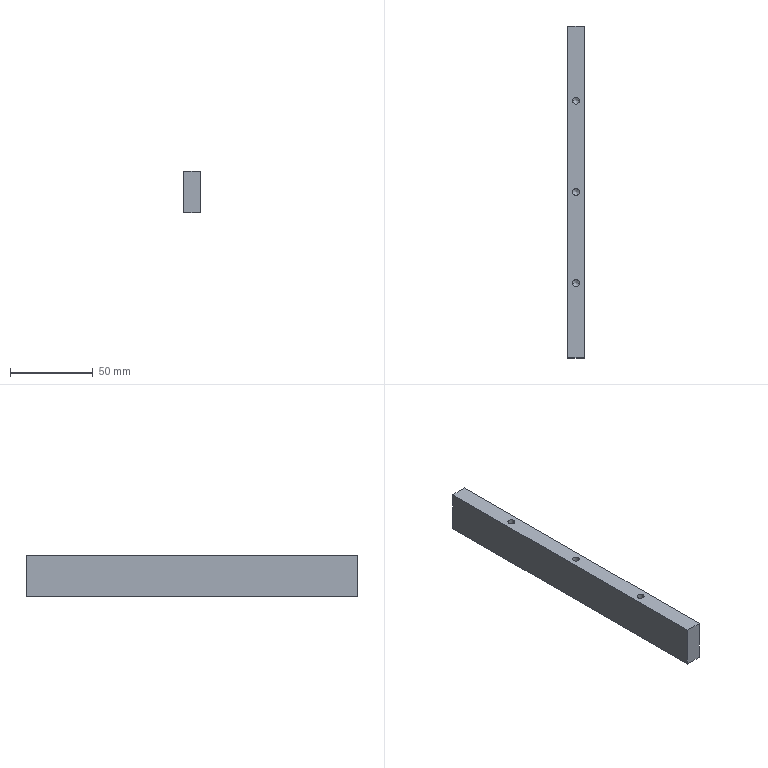Component | SolidWorks | P-SLJ-001-001-1 | 1 solid | 18 faces | box 10 x 200 x 25 mm | volume 49401 mm3 | cylinder 6 | cone 6 | plane 6 | commonest cylinder face diameters 4.2 x6 | material 45#
build123d program:
from build123d import *

# Parameters (mm, degrees)
SKETCH1_W             = 10
SKETCH1_H             = 200
EXTRUDE1_DEPTH        = 12.5
M5_TAPPED_HOLE1_D     = 4.2
M5_TAPPED_HOLE1_DEPTH = 14
M5_TAPPED_HOLE1_TIP   = 1.262


with BuildPart() as part:
    # Sketch1 → Extrude1 (new, symmetric)
    with BuildSketch(Plane(origin=(0, 0, 0), x_dir=(0, 0, -1), z_dir=(1, 0, 0))):
        Rectangle(SKETCH1_W, SKETCH1_H)
    extrude(amount=EXTRUDE1_DEPTH, both=True)

    # M5 Tapped Hole1
    with Locations(Plane.ZY.offset(12.5)):
        with Locations((0, 55), (0, 0), (0, -55)):
            Hole(M5_TAPPED_HOLE1_D / 2, depth=M5_TAPPED_HOLE1_DEPTH)
            with Locations((0, 0, -(M5_TAPPED_HOLE1_DEPTH + M5_TAPPED_HOLE1_TIP / 2))):  # 118° drill point
                Cone(0, M5_TAPPED_HOLE1_D / 2, M5_TAPPED_HOLE1_TIP, mode=Mode.SUBTRACT)


solid = part.part

# Placed as in the assembly
solid = solid.moved(Location((221.5, 0, 1213.134), (0, 90, 0)))
STEP:
#1=COLOUR_RGB('',0.7922,0.8196,0.9333);
#2=FILL_AREA_STYLE_COLOUR('',#1);
#3=FILL_AREA_STYLE('',(#2));
#4=SURFACE_STYLE_FILL_AREA(#3);
#5=SURFACE_SIDE_STYLE('',(#4));
#6=SURFACE_STYLE_USAGE(.BOTH.,#5);
#7=PRESENTATION_STYLE_ASSIGNMENT((#6));
#8=CARTESIAN_POINT('',(8.638,2.165,47.702));
#9=VERTEX_POINT('',#8);
#10=CARTESIAN_POINT('',(8.803,2.165,47.702));
#11=VERTEX_POINT('',#10);
#12=CARTESIAN_POINT('',(8.72,2.165,47.702));
#13=DIRECTION('',(0.,0.,1.));
#14=DIRECTION('',(1.,0.,0.));
#15=AXIS2_PLACEMENT_3D('',#12,#13,#14);
#16=CIRCLE('',#15,0.08268);
#17=EDGE_CURVE('',#9,#11,#16,.T.);
#18=ORIENTED_EDGE('',*,*,#17,.F.);
#19=CARTESIAN_POINT('',(8.638,2.165,48.253));
#20=VERTEX_POINT('',#19);
#21=CARTESIAN_POINT('',(8.638,2.165,48.253));
#22=DIRECTION('',(0.,0.,1.));
#23=VECTOR('',#22,39.37);
#24=LINE('',#21,#23);
#25=EDGE_CURVE('',#9,#20,#24,.T.);
#26=ORIENTED_EDGE('',*,*,#25,.T.);
#27=CARTESIAN_POINT('',(8.803,2.165,48.253));
#28=VERTEX_POINT('',#27);
#29=CARTESIAN_POINT('',(8.72,2.165,48.253));
#30=DIRECTION('',(0.,0.,1.));
#31=DIRECTION('',(1.,0.,0.));
#32=AXIS2_PLACEMENT_3D('',#29,#30,#31);
#33=CIRCLE('',#32,0.08268);
#34=EDGE_CURVE('',#20,#28,#33,.T.);
#35=ORIENTED_EDGE('',*,*,#34,.T.);
#36=CARTESIAN_POINT('',(8.803,2.165,48.253));
#37=DIRECTION('',(0.,0.,1.));
#38=VECTOR('',#37,39.37);
#39=LINE('',#36,#38);
#40=EDGE_CURVE('',#11,#28,#39,.T.);
#41=ORIENTED_EDGE('',*,*,#40,.F.);
#42=EDGE_LOOP('',(#18,#26,#35,#41));
#43=FACE_OUTER_BOUND('',#42,.T.);
#44=CARTESIAN_POINT('',(8.72,2.165,48.253));
#45=DIRECTION('',(0.,0.,1.));
#46=DIRECTION('',(1.,0.,0.));
#47=AXIS2_PLACEMENT_3D('',#44,#45,#46);
#48=CYLINDRICAL_SURFACE('',#47,0.08268);
#49=ADVANCED_FACE('',(#43),#48,.F.);
#50=CARTESIAN_POINT('',(8.72,2.165,47.652));
#51=VERTEX_POINT('',#50);
#52=CARTESIAN_POINT('',(8.803,2.165,47.702));
#53=DIRECTION('',(0.8572,-0.,0.515));
#54=VECTOR('',#53,39.37);
#55=LINE('',#52,#54);
#56=EDGE_CURVE('',#51,#11,#55,.T.);
#57=ORIENTED_EDGE('',*,*,#56,.F.);
#58=CARTESIAN_POINT('',(8.638,2.165,47.702));
#59=DIRECTION('',(-0.8572,0.,0.515));
#60=VECTOR('',#59,39.37);
#61=LINE('',#58,#60);
#62=EDGE_CURVE('',#51,#9,#61,.T.);
#63=ORIENTED_EDGE('',*,*,#62,.T.);
#64=ORIENTED_EDGE('',*,*,#17,.T.);
#65=EDGE_LOOP('',(#57,#63,#64));
#66=FACE_OUTER_BOUND('',#65,.T.);
#67=CARTESIAN_POINT('',(8.72,2.165,47.702));
#68=DIRECTION('',(0.,0.,1.));
#69=DIRECTION('',(1.,0.,0.));
#70=AXIS2_PLACEMENT_3D('',#67,#68,#69);
#71=CONICAL_SURFACE('',#70,0.08268,1.03);
#72=ADVANCED_FACE('',(#66),#71,.F.);
#73=CARTESIAN_POINT('',(8.638,-0.,47.702));
#74=VERTEX_POINT('',#73);
#75=CARTESIAN_POINT('',(8.803,-0.,47.702));
#76=VERTEX_POINT('',#75);
#77=CARTESIAN_POINT('',(8.72,-0.,47.702));
#78=DIRECTION('',(0.,0.,1.));
#79=DIRECTION('',(1.,-0.,0.));
#80=AXIS2_PLACEMENT_3D('',#77,#78,#79);
#81=CIRCLE('',#80,0.08268);
#82=EDGE_CURVE('',#74,#76,#81,.T.);
#83=ORIENTED_EDGE('',*,*,#82,.F.);
#84=CARTESIAN_POINT('',(8.638,-0.,48.253));
#85=VERTEX_POINT('',#84);
#86=CARTESIAN_POINT('',(8.638,-0.,48.253));
#87=DIRECTION('',(0.,0.,1.));
#88=VECTOR('',#87,39.37);
#89=LINE('',#86,#88);
#90=EDGE_CURVE('',#74,#85,#89,.T.);
#91=ORIENTED_EDGE('',*,*,#90,.T.);
#92=CARTESIAN_POINT('',(8.803,-0.,48.253));
#93=VERTEX_POINT('',#92);
#94=CARTESIAN_POINT('',(8.72,-0.,48.253));
#95=DIRECTION('',(0.,0.,1.));
#96=DIRECTION('',(1.,-0.,0.));
#97=AXIS2_PLACEMENT_3D('',#94,#95,#96);
#98=CIRCLE('',#97,0.08268);
#99=EDGE_CURVE('',#85,#93,#98,.T.);
#100=ORIENTED_EDGE('',*,*,#99,.T.);
#101=CARTESIAN_POINT('',(8.803,-0.,48.253));
#102=DIRECTION('',(0.,0.,1.));
#103=VECTOR('',#102,39.37);
#104=LINE('',#101,#103);
#105=EDGE_CURVE('',#76,#93,#104,.T.);
#106=ORIENTED_EDGE('',*,*,#105,.F.);
#107=EDGE_LOOP('',(#83,#91,#100,#106));
#108=FACE_OUTER_BOUND('',#107,.T.);
#109=CARTESIAN_POINT('',(8.72,-0.,48.253));
#110=DIRECTION('',(0.,0.,1.));
#111=DIRECTION('',(1.,-0.,0.));
#112=AXIS2_PLACEMENT_3D('',#109,#110,#111);
#113=CYLINDRICAL_SURFACE('',#112,0.08268);
#114=ADVANCED_FACE('',(#108),#113,.F.);
#115=CARTESIAN_POINT('',(8.72,-0.,47.652));
#116=VERTEX_POINT('',#115);
#117=CARTESIAN_POINT('',(8.803,-0.,47.702));
#118=DIRECTION('',(0.8572,-0.,0.515));
#119=VECTOR('',#118,39.37);
#120=LINE('',#117,#119);
#121=EDGE_CURVE('',#116,#76,#120,.T.);
#122=ORIENTED_EDGE('',*,*,#121,.F.);
#123=CARTESIAN_POINT('',(8.638,-0.,47.702));
#124=DIRECTION('',(-0.8572,0.,0.515));
#125=VECTOR('',#124,39.37);
#126=LINE('',#123,#125);
#127=EDGE_CURVE('',#116,#74,#126,.T.);
#128=ORIENTED_EDGE('',*,*,#127,.T.);
#129=ORIENTED_EDGE('',*,*,#82,.T.);
#130=EDGE_LOOP('',(#122,#128,#129));
#131=FACE_OUTER_BOUND('',#130,.T.);
#132=CARTESIAN_POINT('',(8.72,-0.,47.702));
#133=DIRECTION('',(0.,0.,1.));
#134=DIRECTION('',(1.,-0.,0.));
#135=AXIS2_PLACEMENT_3D('',#132,#133,#134);
#136=CONICAL_SURFACE('',#135,0.08268,1.03);
#137=ADVANCED_FACE('',(#131),#136,.F.);
#138=CARTESIAN_POINT('',(8.638,-2.165,47.702));
#139=VERTEX_POINT('',#138);
#140=CARTESIAN_POINT('',(8.803,-2.165,47.702));
#141=VERTEX_POINT('',#140);
#142=CARTESIAN_POINT('',(8.72,-2.165,47.702));
#143=DIRECTION('',(0.,0.,1.));
#144=DIRECTION('',(1.,0.,0.));
#145=AXIS2_PLACEMENT_3D('',#142,#143,#144);
#146=CIRCLE('',#145,0.08268);
#147=EDGE_CURVE('',#139,#141,#146,.T.);
#148=ORIENTED_EDGE('',*,*,#147,.F.);
#149=CARTESIAN_POINT('',(8.638,-2.165,48.253));
#150=VERTEX_POINT('',#149);
#151=CARTESIAN_POINT('',(8.638,-2.165,48.253));
#152=DIRECTION('',(0.,0.,1.));
#153=VECTOR('',#152,39.37);
#154=LINE('',#151,#153);
#155=EDGE_CURVE('',#139,#150,#154,.T.);
#156=ORIENTED_EDGE('',*,*,#155,.T.);
#157=CARTESIAN_POINT('',(8.803,-2.165,48.253));
#158=VERTEX_POINT('',#157);
#159=CARTESIAN_POINT('',(8.72,-2.165,48.253));
#160=DIRECTION('',(0.,0.,1.));
#161=DIRECTION('',(1.,0.,0.));
#162=AXIS2_PLACEMENT_3D('',#159,#160,#161);
#163=CIRCLE('',#162,0.08268);
#164=EDGE_CURVE('',#150,#158,#163,.T.);
#165=ORIENTED_EDGE('',*,*,#164,.T.);
#166=CARTESIAN_POINT('',(8.803,-2.165,48.253));
#167=DIRECTION('',(0.,0.,1.));
#168=VECTOR('',#167,39.37);
#169=LINE('',#166,#168);
#170=EDGE_CURVE('',#141,#158,#169,.T.);
#171=ORIENTED_EDGE('',*,*,#170,.F.);
#172=EDGE_LOOP('',(#148,#156,#165,#171));
#173=FACE_OUTER_BOUND('',#172,.T.);
#174=CARTESIAN_POINT('',(8.72,-2.165,48.253));
#175=DIRECTION('',(0.,0.,1.));
#176=DIRECTION('',(1.,0.,0.));
#177=AXIS2_PLACEMENT_3D('',#174,#175,#176);
#178=CYLINDRICAL_SURFACE('',#177,0.08268);
#179=ADVANCED_FACE('',(#173),#178,.F.);
#180=CARTESIAN_POINT('',(8.72,-2.165,47.652));
#181=VERTEX_POINT('',#180);
#182=CARTESIAN_POINT('',(8.803,-2.165,47.702));
#183=DIRECTION('',(0.8572,-0.,0.515));
#184=VECTOR('',#183,39.37);
#185=LINE('',#182,#184);
#186=EDGE_CURVE('',#181,#141,#185,.T.);
#187=ORIENTED_EDGE('',*,*,#186,.F.);
#188=CARTESIAN_POINT('',(8.638,-2.165,47.702));
#189=DIRECTION('',(-0.8572,0.,0.515));
#190=VECTOR('',#189,39.37);
#191=LINE('',#188,#190);
#192=EDGE_CURVE('',#181,#139,#191,.T.);
#193=ORIENTED_EDGE('',*,*,#192,.T.);
#194=ORIENTED_EDGE('',*,*,#147,.T.);
#195=EDGE_LOOP('',(#187,#193,#194));
#196=FACE_OUTER_BOUND('',#195,.T.);
#197=CARTESIAN_POINT('',(8.72,-2.165,47.702));
#198=DIRECTION('',(0.,0.,1.));
#199=DIRECTION('',(1.,0.,0.));
#200=AXIS2_PLACEMENT_3D('',#197,#198,#199);
#201=CONICAL_SURFACE('',#200,0.08268,1.03);
#202=ADVANCED_FACE('',(#196),#201,.F.);
#203=CARTESIAN_POINT('',(8.524,-3.937,48.253));
#204=VERTEX_POINT('',#203);
#205=CARTESIAN_POINT('',(8.524,3.937,48.253));
#206=VERTEX_POINT('',#205);
#207=CARTESIAN_POINT('',(8.524,-3.937,48.253));
#208=DIRECTION('',(0.,1.,0.));
#209=VECTOR('',#208,39.37);
#210=LINE('',#207,#209);
#211=EDGE_CURVE('',#204,#206,#210,.T.);
#212=ORIENTED_EDGE('',*,*,#211,.T.);
#213=CARTESIAN_POINT('',(8.524,3.937,47.269));
#214=VERTEX_POINT('',#213);
#215=CARTESIAN_POINT('',(8.524,3.937,47.269));
#216=DIRECTION('',(0.,0.,1.));
#217=VECTOR('',#216,39.37);
#218=LINE('',#215,#217);
#219=EDGE_CURVE('',#214,#206,#218,.T.);
#220=ORIENTED_EDGE('',*,*,#219,.F.);
#221=CARTESIAN_POINT('',(8.524,-3.937,47.269));
#222=VERTEX_POINT('',#221);
#223=CARTESIAN_POINT('',(8.524,-3.937,47.269));
#224=DIRECTION('',(0.,1.,0.));
#225=VECTOR('',#224,39.37);
#226=LINE('',#223,#225);
#227=EDGE_CURVE('',#222,#214,#226,.T.);
#228=ORIENTED_EDGE('',*,*,#227,.F.);
#229=CARTESIAN_POINT('',(8.524,-3.937,47.269));
#230=DIRECTION('',(0.,0.,1.));
#231=VECTOR('',#230,39.37);
#232=LINE('',#229,#231);
#233=EDGE_CURVE('',#222,#204,#232,.T.);
#234=ORIENTED_EDGE('',*,*,#233,.T.);
#235=EDGE_LOOP('',(#212,#220,#228,#234));
#236=FACE_OUTER_BOUND('',#235,.T.);
#237=CARTESIAN_POINT('',(8.524,-3.937,47.269));
#238=DIRECTION('',(1.,-0.,0.));
#239=DIRECTION('',(0.,0.,-1.));
#240=AXIS2_PLACEMENT_3D('',#237,#238,#239);
#241=PLANE('',#240);
#242=ADVANCED_FACE('',(#236),#241,.F.);
#243=CARTESIAN_POINT('',(8.917,3.937,48.253));
#244=VERTEX_POINT('',#243);
#245=CARTESIAN_POINT('',(8.917,3.937,48.253));
#246=DIRECTION('',(1.,-0.,0.));
#247=VECTOR('',#246,39.37);
#248=LINE('',#245,#247);
#249=EDGE_CURVE('',#206,#244,#248,.T.);
#250=ORIENTED_EDGE('',*,*,#249,.T.);
#251=CARTESIAN_POINT('',(8.917,3.937,47.269));
#252=VERTEX_POINT('',#251);
#253=CARTESIAN_POINT('',(8.917,3.937,47.269));
#254=DIRECTION('',(0.,0.,1.));
#255=VECTOR('',#254,39.37);
#256=LINE('',#253,#255);
#257=EDGE_CURVE('',#252,#244,#256,.T.);
#258=ORIENTED_EDGE('',*,*,#257,.F.);
#259=CARTESIAN_POINT('',(8.917,3.937,47.269));
#260=DIRECTION('',(1.,-0.,0.));
#261=VECTOR('',#260,39.37);
#262=LINE('',#259,#261);
#263=EDGE_CURVE('',#214,#252,#262,.T.);
#264=ORIENTED_EDGE('',*,*,#263,.F.);
#265=ORIENTED_EDGE('',*,*,#219,.T.);
#266=EDGE_LOOP('',(#250,#258,#264,#265));
#267=FACE_OUTER_BOUND('',#266,.T.);
#268=CARTESIAN_POINT('',(8.917,3.937,47.269));
#269=DIRECTION('',(-0.,-1.,0.));
#270=DIRECTION('',(-1.,0.,0.));
#271=AXIS2_PLACEMENT_3D('',#268,#269,#270);
#272=PLANE('',#271);
#273=ADVANCED_FACE('',(#267),#272,.F.);
#274=CARTESIAN_POINT('',(8.917,-3.937,48.253));
#275=VERTEX_POINT('',#274);
#276=CARTESIAN_POINT('',(8.917,-3.937,48.253));
#277=DIRECTION('',(-0.,-1.,0.));
#278=VECTOR('',#277,39.37);
#279=LINE('',#276,#278);
#280=EDGE_CURVE('',#244,#275,#279,.T.);
#281=ORIENTED_EDGE('',*,*,#280,.T.);
#282=CARTESIAN_POINT('',(8.917,-3.937,47.269));
#283=VERTEX_POINT('',#282);
#284=CARTESIAN_POINT('',(8.917,-3.937,47.269));
#285=DIRECTION('',(0.,0.,1.));
#286=VECTOR('',#285,39.37);
#287=LINE('',#284,#286);
#288=EDGE_CURVE('',#283,#275,#287,.T.);
#289=ORIENTED_EDGE('',*,*,#288,.F.);
#290=CARTESIAN_POINT('',(8.917,-3.937,47.269));
#291=DIRECTION('',(-0.,-1.,0.));
#292=VECTOR('',#291,39.37);
#293=LINE('',#290,#292);
#294=EDGE_CURVE('',#252,#283,#293,.T.);
#295=ORIENTED_EDGE('',*,*,#294,.F.);
#296=ORIENTED_EDGE('',*,*,#257,.T.);
#297=EDGE_LOOP('',(#281,#289,#295,#296));
#298=FACE_OUTER_BOUND('',#297,.T.);
#299=CARTESIAN_POINT('',(8.917,-3.937,47.269));
#300=DIRECTION('',(-1.,0.,0.));
#301=DIRECTION('',(0.,0.,1.));
#302=AXIS2_PLACEMENT_3D('',#299,#300,#301);
#303=PLANE('',#302);
#304=ADVANCED_FACE('',(#298),#303,.F.);
#305=CARTESIAN_POINT('',(8.917,-3.937,48.253));
#306=DIRECTION('',(-1.,0.,0.));
#307=VECTOR('',#306,39.37);
#308=LINE('',#305,#307);
#309=EDGE_CURVE('',#275,#204,#308,.T.);
#310=ORIENTED_EDGE('',*,*,#309,.T.);
#311=ORIENTED_EDGE('',*,*,#233,.F.);
#312=CARTESIAN_POINT('',(8.917,-3.937,47.269));
#313=DIRECTION('',(-1.,0.,0.));
#314=VECTOR('',#313,39.37);
#315=LINE('',#312,#314);
#316=EDGE_CURVE('',#283,#222,#315,.T.);
#317=ORIENTED_EDGE('',*,*,#316,.F.);
#318=ORIENTED_EDGE('',*,*,#288,.T.);
#319=EDGE_LOOP('',(#310,#311,#317,#318));
#320=FACE_OUTER_BOUND('',#319,.T.);
#321=CARTESIAN_POINT('',(8.917,-3.937,47.269));
#322=DIRECTION('',(0.,1.,0.));
#323=DIRECTION('',(1.,-0.,0.));
#324=AXIS2_PLACEMENT_3D('',#321,#322,#323);
#325=PLANE('',#324);
#326=ADVANCED_FACE('',(#320),#325,.F.);
#327=ORIENTED_EDGE('',*,*,#227,.T.);
#328=ORIENTED_EDGE('',*,*,#263,.T.);
#329=ORIENTED_EDGE('',*,*,#294,.T.);
#330=ORIENTED_EDGE('',*,*,#316,.T.);
#331=EDGE_LOOP('',(#327,#328,#329,#330));
#332=FACE_OUTER_BOUND('',#331,.T.);
#333=CARTESIAN_POINT('',(8.72,-0.,47.269));
#334=DIRECTION('',(0.,0.,1.));
#335=DIRECTION('',(1.,-0.,0.));
#336=AXIS2_PLACEMENT_3D('',#333,#334,#335);
#337=PLANE('',#336);
#338=ADVANCED_FACE('',(#332),#337,.F.);
#339=CARTESIAN_POINT('',(8.72,2.165,48.253));
#340=DIRECTION('',(0.,0.,1.));
#341=DIRECTION('',(1.,0.,0.));
#342=AXIS2_PLACEMENT_3D('',#339,#340,#341);
#343=CIRCLE('',#342,0.08268);
#344=EDGE_CURVE('',#28,#20,#343,.T.);
#345=ORIENTED_EDGE('',*,*,#344,.F.);
#346=ORIENTED_EDGE('',*,*,#34,.F.);
#347=EDGE_LOOP('',(#345,#346));
#348=FACE_BOUND('',#347,.T.);
#349=CARTESIAN_POINT('',(8.72,-0.,48.253));
#350=DIRECTION('',(0.,0.,1.));
#351=DIRECTION('',(1.,-0.,0.));
#352=AXIS2_PLACEMENT_3D('',#349,#350,#351);
#353=CIRCLE('',#352,0.08268);
#354=EDGE_CURVE('',#93,#85,#353,.T.);
#355=ORIENTED_EDGE('',*,*,#354,.F.);
#356=ORIENTED_EDGE('',*,*,#99,.F.);
#357=EDGE_LOOP('',(#355,#356));
#358=FACE_BOUND('',#357,.T.);
#359=CARTESIAN_POINT('',(8.72,-2.165,48.253));
#360=DIRECTION('',(0.,0.,1.));
#361=DIRECTION('',(1.,0.,0.));
#362=AXIS2_PLACEMENT_3D('',#359,#360,#361);
#363=CIRCLE('',#362,0.08268);
#364=EDGE_CURVE('',#158,#150,#363,.T.);
#365=ORIENTED_EDGE('',*,*,#364,.F.);
#366=ORIENTED_EDGE('',*,*,#164,.F.);
#367=EDGE_LOOP('',(#365,#366));
#368=FACE_BOUND('',#367,.T.);
#369=ORIENTED_EDGE('',*,*,#211,.F.);
#370=ORIENTED_EDGE('',*,*,#309,.F.);
#371=ORIENTED_EDGE('',*,*,#280,.F.);
#372=ORIENTED_EDGE('',*,*,#249,.F.);
#373=EDGE_LOOP('',(#369,#370,#371,#372));
#374=FACE_OUTER_BOUND('',#373,.T.);
#375=CARTESIAN_POINT('',(8.72,-0.,48.253));
#376=DIRECTION('',(0.,0.,1.));
#377=DIRECTION('',(1.,-0.,0.));
#378=AXIS2_PLACEMENT_3D('',#375,#376,#377);
#379=PLANE('',#378);
#380=ADVANCED_FACE('',(#348,#358,#368,#374),#379,.T.);
#381=ORIENTED_EDGE('',*,*,#192,.F.);
#382=ORIENTED_EDGE('',*,*,#186,.T.);
#383=CARTESIAN_POINT('',(8.72,-2.165,47.702));
#384=DIRECTION('',(0.,0.,1.));
#385=DIRECTION('',(1.,0.,0.));
#386=AXIS2_PLACEMENT_3D('',#383,#384,#385);
#387=CIRCLE('',#386,0.08268);
#388=EDGE_CURVE('',#141,#139,#387,.T.);
#389=ORIENTED_EDGE('',*,*,#388,.T.);
#390=EDGE_LOOP('',(#381,#382,#389));
#391=FACE_OUTER_BOUND('',#390,.T.);
#392=CARTESIAN_POINT('',(8.72,-2.165,47.702));
#393=DIRECTION('',(0.,0.,1.));
#394=DIRECTION('',(1.,0.,0.));
#395=AXIS2_PLACEMENT_3D('',#392,#393,#394);
#396=CONICAL_SURFACE('',#395,0.08268,1.03);
#397=ADVANCED_FACE('',(#391),#396,.F.);
#398=ORIENTED_EDGE('',*,*,#155,.F.);
#399=ORIENTED_EDGE('',*,*,#388,.F.);
#400=ORIENTED_EDGE('',*,*,#170,.T.);
#401=ORIENTED_EDGE('',*,*,#364,.T.);
#402=EDGE_LOOP('',(#398,#399,#400,#401));
#403=FACE_OUTER_BOUND('',#402,.T.);
#404=CARTESIAN_POINT('',(8.72,-2.165,48.253));
#405=DIRECTION('',(0.,0.,1.));
#406=DIRECTION('',(1.,0.,0.));
#407=AXIS2_PLACEMENT_3D('',#404,#405,#406);
#408=CYLINDRICAL_SURFACE('',#407,0.08268);
#409=ADVANCED_FACE('',(#403),#408,.F.);
#410=ORIENTED_EDGE('',*,*,#127,.F.);
#411=ORIENTED_EDGE('',*,*,#121,.T.);
#412=CARTESIAN_POINT('',(8.72,-0.,47.702));
#413=DIRECTION('',(0.,0.,1.));
#414=DIRECTION('',(1.,-0.,0.));
#415=AXIS2_PLACEMENT_3D('',#412,#413,#414);
#416=CIRCLE('',#415,0.08268);
#417=EDGE_CURVE('',#76,#74,#416,.T.);
#418=ORIENTED_EDGE('',*,*,#417,.T.);
#419=EDGE_LOOP('',(#410,#411,#418));
#420=FACE_OUTER_BOUND('',#419,.T.);
#421=CARTESIAN_POINT('',(8.72,-0.,47.702));
#422=DIRECTION('',(0.,0.,1.));
#423=DIRECTION('',(1.,-0.,0.));
#424=AXIS2_PLACEMENT_3D('',#421,#422,#423);
#425=CONICAL_SURFACE('',#424,0.08268,1.03);
#426=ADVANCED_FACE('',(#420),#425,.F.);
#427=ORIENTED_EDGE('',*,*,#90,.F.);
#428=ORIENTED_EDGE('',*,*,#417,.F.);
#429=ORIENTED_EDGE('',*,*,#105,.T.);
#430=ORIENTED_EDGE('',*,*,#354,.T.);
#431=EDGE_LOOP('',(#427,#428,#429,#430));
#432=FACE_OUTER_BOUND('',#431,.T.);
#433=CARTESIAN_POINT('',(8.72,-0.,48.253));
#434=DIRECTION('',(0.,0.,1.));
#435=DIRECTION('',(1.,-0.,0.));
#436=AXIS2_PLACEMENT_3D('',#433,#434,#435);
#437=CYLINDRICAL_SURFACE('',#436,0.08268);
#438=ADVANCED_FACE('',(#432),#437,.F.);
#439=ORIENTED_EDGE('',*,*,#62,.F.);
#440=ORIENTED_EDGE('',*,*,#56,.T.);
#441=CARTESIAN_POINT('',(8.72,2.165,47.702));
#442=DIRECTION('',(0.,0.,1.));
#443=DIRECTION('',(1.,0.,0.));
#444=AXIS2_PLACEMENT_3D('',#441,#442,#443);
#445=CIRCLE('',#444,0.08268);
#446=EDGE_CURVE('',#11,#9,#445,.T.);
#447=ORIENTED_EDGE('',*,*,#446,.T.);
#448=EDGE_LOOP('',(#439,#440,#447));
#449=FACE_OUTER_BOUND('',#448,.T.);
#450=CARTESIAN_POINT('',(8.72,2.165,47.702));
#451=DIRECTION('',(0.,0.,1.));
#452=DIRECTION('',(1.,0.,0.));
#453=AXIS2_PLACEMENT_3D('',#450,#451,#452);
#454=CONICAL_SURFACE('',#453,0.08268,1.03);
#455=ADVANCED_FACE('',(#449),#454,.F.);
#456=ORIENTED_EDGE('',*,*,#25,.F.);
#457=ORIENTED_EDGE('',*,*,#446,.F.);
#458=ORIENTED_EDGE('',*,*,#40,.T.);
#459=ORIENTED_EDGE('',*,*,#344,.T.);
#460=EDGE_LOOP('',(#456,#457,#458,#459));
#461=FACE_OUTER_BOUND('',#460,.T.);
#462=CARTESIAN_POINT('',(8.72,2.165,48.253));
#463=DIRECTION('',(0.,0.,1.));
#464=DIRECTION('',(1.,0.,0.));
#465=AXIS2_PLACEMENT_3D('',#462,#463,#464);
#466=CYLINDRICAL_SURFACE('',#465,0.08268);
#467=ADVANCED_FACE('',(#461),#466,.F.);
#468=CLOSED_SHELL('',(#49,#72,#114,#137,#179,#202,#242,#273,#304,#326,#338,#380,#397,#409,#426,#438,#455,#467));
#469=MANIFOLD_SOLID_BREP('',#468);
#470=STYLED_ITEM('',(#7),#469);
#471=PRESENTATION_LAYER_ASSIGNMENT('','',(#470));
#472=CARTESIAN_POINT('',(0.,0.,0.));
#473=DIRECTION('',(0.,0.,1.));
#474=DIRECTION('',(1.,0.,0.));
#475=AXIS2_PLACEMENT_3D('',#472,#473,#474);
#476=(LENGTH_UNIT()NAMED_UNIT(*)SI_UNIT($,.METRE.));
#477=LENGTH_MEASURE_WITH_UNIT(LENGTH_MEASURE(0.0254),#476);
#478=DIMENSIONAL_EXPONENTS(1.,0.,0.,0.,0.,0.,0.);
#479=(CONVERSION_BASED_UNIT('',#477)LENGTH_UNIT()NAMED_UNIT(#478));
#480=UNCERTAINTY_MEASURE_WITH_UNIT(LENGTH_MEASURE(0.00001),#479,'','');
#481=(NAMED_UNIT(*)PLANE_ANGLE_UNIT()SI_UNIT($,.RADIAN.));
#482=(NAMED_UNIT(*)SI_UNIT($,.STERADIAN.)SOLID_ANGLE_UNIT());
#483=(GEOMETRIC_REPRESENTATION_CONTEXT(3)GLOBAL_UNCERTAINTY_ASSIGNED_CONTEXT((#480))GLOBAL_UNIT_ASSIGNED_CONTEXT((#479,#481,#482))REPRESENTATION_CONTEXT('',''));
#484=ADVANCED_BREP_SHAPE_REPRESENTATION('',(#469,#475),#483);
#485=(LENGTH_UNIT()NAMED_UNIT(*)SI_UNIT($,.METRE.));
#486=LENGTH_MEASURE_WITH_UNIT(LENGTH_MEASURE(0.0254),#485);
#487=DIMENSIONAL_EXPONENTS(1.,0.,0.,0.,0.,0.,0.);
#488=(CONVERSION_BASED_UNIT('',#486)LENGTH_UNIT()NAMED_UNIT(#487));
#489=UNCERTAINTY_MEASURE_WITH_UNIT(LENGTH_MEASURE(0.00001),#488,'','');
#490=(NAMED_UNIT(*)PLANE_ANGLE_UNIT()SI_UNIT($,.RADIAN.));
#491=(NAMED_UNIT(*)SI_UNIT($,.STERADIAN.)SOLID_ANGLE_UNIT());
#492=(GEOMETRIC_REPRESENTATION_CONTEXT(3)GLOBAL_UNCERTAINTY_ASSIGNED_CONTEXT((#489))GLOBAL_UNIT_ASSIGNED_CONTEXT((#488,#490,#491))REPRESENTATION_CONTEXT('',''));
#493=MECHANICAL_DESIGN_GEOMETRIC_PRESENTATION_REPRESENTATION('',(#470),#492);